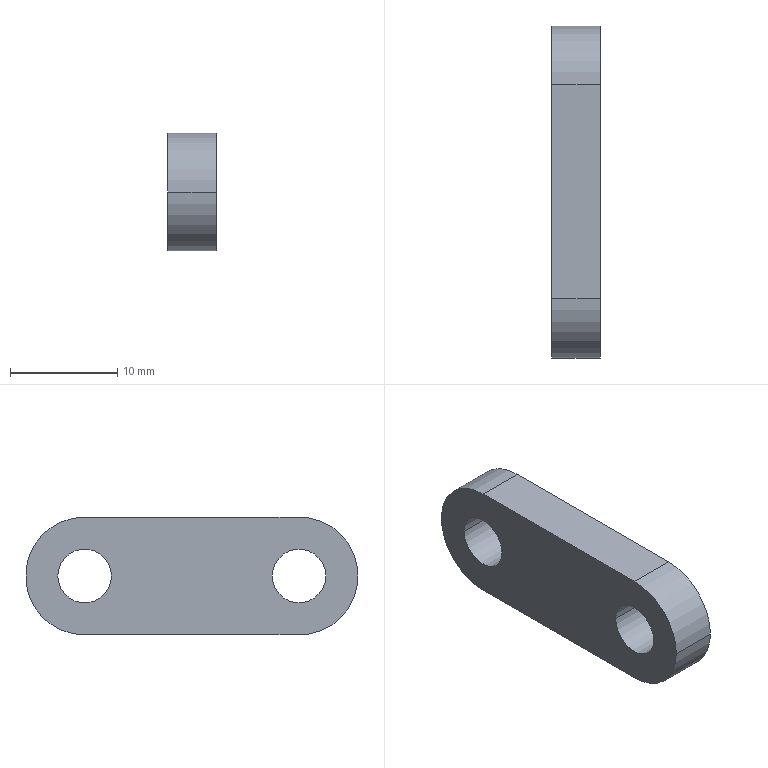Component | SolidWorks | LeverHydraulicRod22-1_HLKA-22_-0-2 | 1 solid | 11 faces | box 4.5 x 31 x 11 mm | volume 1241 mm3 | cylinder 7 | plane 4 | commonest cylinder face diameters 5 x4 11 x3
STEP:
#1=CARTESIAN_POINT('',(-2.288,4.392,-3.051));
#2=VERTEX_POINT('',#1);
#3=CARTESIAN_POINT('',(-2.288,4.588,-3.051));
#4=VERTEX_POINT('',#3);
#5=CARTESIAN_POINT('',(-2.288,4.49,-3.051));
#6=DIRECTION('',(1.,0.,0.));
#7=DIRECTION('',(0.,1.,0.));
#8=AXIS2_PLACEMENT_3D('',#5,#6,#7);
#9=CIRCLE('',#8,0.09843);
#10=EDGE_CURVE('',#2,#4,#9,.T.);
#11=ORIENTED_EDGE('',*,*,#10,.T.);
#12=CARTESIAN_POINT('',(-2.465,4.588,-3.051));
#13=VERTEX_POINT('',#12);
#14=CARTESIAN_POINT('',(-2.288,4.588,-3.051));
#15=DIRECTION('',(-1.,-0.,-0.));
#16=VECTOR('',#15,39.37);
#17=LINE('',#14,#16);
#18=EDGE_CURVE('',#4,#13,#17,.T.);
#19=ORIENTED_EDGE('',*,*,#18,.T.);
#20=CARTESIAN_POINT('',(-2.465,4.392,-3.051));
#21=VERTEX_POINT('',#20);
#22=CARTESIAN_POINT('',(-2.465,4.49,-3.051));
#23=DIRECTION('',(1.,0.,0.));
#24=DIRECTION('',(0.,1.,0.));
#25=AXIS2_PLACEMENT_3D('',#22,#23,#24);
#26=CIRCLE('',#25,0.09843);
#27=EDGE_CURVE('',#21,#13,#26,.T.);
#28=ORIENTED_EDGE('',*,*,#27,.F.);
#29=CARTESIAN_POINT('',(-2.288,4.392,-3.051));
#30=DIRECTION('',(-1.,-0.,-0.));
#31=VECTOR('',#30,39.37);
#32=LINE('',#29,#31);
#33=EDGE_CURVE('',#2,#21,#32,.T.);
#34=ORIENTED_EDGE('',*,*,#33,.F.);
#35=EDGE_LOOP('',(#11,#19,#28,#34));
#36=FACE_OUTER_BOUND('',#35,.T.);
#37=CARTESIAN_POINT('',(-2.288,4.49,-3.051));
#38=DIRECTION('',(-1.,-0.,-0.));
#39=DIRECTION('',(0.,-1.,0.));
#40=AXIS2_PLACEMENT_3D('',#37,#38,#39);
#41=CYLINDRICAL_SURFACE('',#40,0.09843);
#42=ADVANCED_FACE('',(#36),#41,.F.);
#43=CARTESIAN_POINT('',(-2.288,3.604,-3.051));
#44=VERTEX_POINT('',#43);
#45=CARTESIAN_POINT('',(-2.288,3.801,-3.051));
#46=VERTEX_POINT('',#45);
#47=CARTESIAN_POINT('',(-2.288,3.703,-3.051));
#48=DIRECTION('',(1.,0.,0.));
#49=DIRECTION('',(0.,1.,0.));
#50=AXIS2_PLACEMENT_3D('',#47,#48,#49);
#51=CIRCLE('',#50,0.09843);
#52=EDGE_CURVE('',#44,#46,#51,.T.);
#53=ORIENTED_EDGE('',*,*,#52,.T.);
#54=CARTESIAN_POINT('',(-2.465,3.801,-3.051));
#55=VERTEX_POINT('',#54);
#56=CARTESIAN_POINT('',(-2.288,3.801,-3.051));
#57=DIRECTION('',(-1.,-0.,-0.));
#58=VECTOR('',#57,39.37);
#59=LINE('',#56,#58);
#60=EDGE_CURVE('',#46,#55,#59,.T.);
#61=ORIENTED_EDGE('',*,*,#60,.T.);
#62=CARTESIAN_POINT('',(-2.465,3.604,-3.051));
#63=VERTEX_POINT('',#62);
#64=CARTESIAN_POINT('',(-2.465,3.703,-3.051));
#65=DIRECTION('',(1.,0.,0.));
#66=DIRECTION('',(0.,1.,0.));
#67=AXIS2_PLACEMENT_3D('',#64,#65,#66);
#68=CIRCLE('',#67,0.09843);
#69=EDGE_CURVE('',#63,#55,#68,.T.);
#70=ORIENTED_EDGE('',*,*,#69,.F.);
#71=CARTESIAN_POINT('',(-2.288,3.604,-3.051));
#72=DIRECTION('',(-1.,-0.,-0.));
#73=VECTOR('',#72,39.37);
#74=LINE('',#71,#73);
#75=EDGE_CURVE('',#44,#63,#74,.T.);
#76=ORIENTED_EDGE('',*,*,#75,.F.);
#77=EDGE_LOOP('',(#53,#61,#70,#76));
#78=FACE_OUTER_BOUND('',#77,.T.);
#79=CARTESIAN_POINT('',(-2.288,3.703,-3.051));
#80=DIRECTION('',(-1.,-0.,-0.));
#81=DIRECTION('',(0.,-1.,0.));
#82=AXIS2_PLACEMENT_3D('',#79,#80,#81);
#83=CYLINDRICAL_SURFACE('',#82,0.09843);
#84=ADVANCED_FACE('',(#78),#83,.F.);
#85=CARTESIAN_POINT('',(-2.288,3.486,-3.051));
#86=VERTEX_POINT('',#85);
#87=CARTESIAN_POINT('',(-2.288,3.703,-3.268));
#88=VERTEX_POINT('',#87);
#89=CARTESIAN_POINT('',(-2.288,3.703,-3.051));
#90=DIRECTION('',(1.,0.,0.));
#91=DIRECTION('',(0.,1.,0.));
#92=AXIS2_PLACEMENT_3D('',#89,#90,#91);
#93=CIRCLE('',#92,0.2165);
#94=EDGE_CURVE('',#86,#88,#93,.T.);
#95=ORIENTED_EDGE('',*,*,#94,.F.);
#96=CARTESIAN_POINT('',(-2.465,3.486,-3.051));
#97=VERTEX_POINT('',#96);
#98=CARTESIAN_POINT('',(-2.288,3.486,-3.051));
#99=DIRECTION('',(-1.,-0.,-0.));
#100=VECTOR('',#99,39.37);
#101=LINE('',#98,#100);
#102=EDGE_CURVE('',#86,#97,#101,.T.);
#103=ORIENTED_EDGE('',*,*,#102,.T.);
#104=CARTESIAN_POINT('',(-2.465,3.703,-3.268));
#105=VERTEX_POINT('',#104);
#106=CARTESIAN_POINT('',(-2.465,3.703,-3.051));
#107=DIRECTION('',(1.,0.,0.));
#108=DIRECTION('',(0.,1.,0.));
#109=AXIS2_PLACEMENT_3D('',#106,#107,#108);
#110=CIRCLE('',#109,0.2165);
#111=EDGE_CURVE('',#97,#105,#110,.T.);
#112=ORIENTED_EDGE('',*,*,#111,.T.);
#113=CARTESIAN_POINT('',(-2.288,3.703,-3.268));
#114=DIRECTION('',(-1.,-0.,-0.));
#115=VECTOR('',#114,39.37);
#116=LINE('',#113,#115);
#117=EDGE_CURVE('',#88,#105,#116,.T.);
#118=ORIENTED_EDGE('',*,*,#117,.F.);
#119=EDGE_LOOP('',(#95,#103,#112,#118));
#120=FACE_OUTER_BOUND('',#119,.T.);
#121=CARTESIAN_POINT('',(-2.288,3.703,-3.051));
#122=DIRECTION('',(-1.,-0.,-0.));
#123=DIRECTION('',(0.,-1.,0.));
#124=AXIS2_PLACEMENT_3D('',#121,#122,#123);
#125=CYLINDRICAL_SURFACE('',#124,0.2165);
#126=ADVANCED_FACE('',(#120),#125,.T.);
#127=CARTESIAN_POINT('',(-2.465,4.49,-2.835));
#128=VERTEX_POINT('',#127);
#129=CARTESIAN_POINT('',(-2.465,3.703,-2.835));
#130=VERTEX_POINT('',#129);
#131=CARTESIAN_POINT('',(-2.465,3.703,-2.835));
#132=DIRECTION('',(-0.,-1.,0.));
#133=VECTOR('',#132,39.37);
#134=LINE('',#131,#133);
#135=EDGE_CURVE('',#128,#130,#134,.T.);
#136=ORIENTED_EDGE('',*,*,#135,.T.);
#137=CARTESIAN_POINT('',(-2.288,3.703,-2.835));
#138=VERTEX_POINT('',#137);
#139=CARTESIAN_POINT('',(-2.288,3.703,-2.835));
#140=DIRECTION('',(-1.,-0.,-0.));
#141=VECTOR('',#140,39.37);
#142=LINE('',#139,#141);
#143=EDGE_CURVE('',#138,#130,#142,.T.);
#144=ORIENTED_EDGE('',*,*,#143,.F.);
#145=CARTESIAN_POINT('',(-2.288,4.49,-2.835));
#146=VERTEX_POINT('',#145);
#147=CARTESIAN_POINT('',(-2.288,3.703,-2.835));
#148=DIRECTION('',(-0.,-1.,0.));
#149=VECTOR('',#148,39.37);
#150=LINE('',#147,#149);
#151=EDGE_CURVE('',#146,#138,#150,.T.);
#152=ORIENTED_EDGE('',*,*,#151,.F.);
#153=CARTESIAN_POINT('',(-2.288,4.49,-2.835));
#154=DIRECTION('',(-1.,-0.,-0.));
#155=VECTOR('',#154,39.37);
#156=LINE('',#153,#155);
#157=EDGE_CURVE('',#146,#128,#156,.T.);
#158=ORIENTED_EDGE('',*,*,#157,.T.);
#159=EDGE_LOOP('',(#136,#144,#152,#158));
#160=FACE_OUTER_BOUND('',#159,.T.);
#161=CARTESIAN_POINT('',(-2.288,3.703,-2.835));
#162=DIRECTION('',(0.,-0.,-1.));
#163=DIRECTION('',(-1.,-0.,-0.));
#164=AXIS2_PLACEMENT_3D('',#161,#162,#163);
#165=PLANE('',#164);
#166=ADVANCED_FACE('',(#160),#165,.F.);
#167=CARTESIAN_POINT('',(-2.465,4.49,-3.268));
#168=VERTEX_POINT('',#167);
#169=CARTESIAN_POINT('',(-2.465,4.49,-3.051));
#170=DIRECTION('',(1.,0.,0.));
#171=DIRECTION('',(0.,1.,0.));
#172=AXIS2_PLACEMENT_3D('',#169,#170,#171);
#173=CIRCLE('',#172,0.2165);
#174=EDGE_CURVE('',#168,#128,#173,.T.);
#175=ORIENTED_EDGE('',*,*,#174,.T.);
#176=ORIENTED_EDGE('',*,*,#157,.F.);
#177=CARTESIAN_POINT('',(-2.288,4.49,-3.268));
#178=VERTEX_POINT('',#177);
#179=CARTESIAN_POINT('',(-2.288,4.49,-3.051));
#180=DIRECTION('',(1.,0.,0.));
#181=DIRECTION('',(0.,1.,0.));
#182=AXIS2_PLACEMENT_3D('',#179,#180,#181);
#183=CIRCLE('',#182,0.2165);
#184=EDGE_CURVE('',#178,#146,#183,.T.);
#185=ORIENTED_EDGE('',*,*,#184,.F.);
#186=CARTESIAN_POINT('',(-2.288,4.49,-3.268));
#187=DIRECTION('',(-1.,-0.,-0.));
#188=VECTOR('',#187,39.37);
#189=LINE('',#186,#188);
#190=EDGE_CURVE('',#178,#168,#189,.T.);
#191=ORIENTED_EDGE('',*,*,#190,.T.);
#192=EDGE_LOOP('',(#175,#176,#185,#191));
#193=FACE_OUTER_BOUND('',#192,.T.);
#194=CARTESIAN_POINT('',(-2.288,4.49,-3.051));
#195=DIRECTION('',(-1.,-0.,-0.));
#196=DIRECTION('',(0.,-1.,0.));
#197=AXIS2_PLACEMENT_3D('',#194,#195,#196);
#198=CYLINDRICAL_SURFACE('',#197,0.2165);
#199=ADVANCED_FACE('',(#193),#198,.T.);
#200=CARTESIAN_POINT('',(-2.465,3.703,-3.268));
#201=DIRECTION('',(0.,1.,-0.));
#202=VECTOR('',#201,39.37);
#203=LINE('',#200,#202);
#204=EDGE_CURVE('',#105,#168,#203,.T.);
#205=ORIENTED_EDGE('',*,*,#204,.T.);
#206=ORIENTED_EDGE('',*,*,#190,.F.);
#207=CARTESIAN_POINT('',(-2.288,3.703,-3.268));
#208=DIRECTION('',(0.,1.,-0.));
#209=VECTOR('',#208,39.37);
#210=LINE('',#207,#209);
#211=EDGE_CURVE('',#88,#178,#210,.T.);
#212=ORIENTED_EDGE('',*,*,#211,.F.);
#213=ORIENTED_EDGE('',*,*,#117,.T.);
#214=EDGE_LOOP('',(#205,#206,#212,#213));
#215=FACE_OUTER_BOUND('',#214,.T.);
#216=CARTESIAN_POINT('',(-2.288,3.703,-3.268));
#217=DIRECTION('',(-0.,0.,1.));
#218=DIRECTION('',(0.,1.,-0.));
#219=AXIS2_PLACEMENT_3D('',#216,#217,#218);
#220=PLANE('',#219);
#221=ADVANCED_FACE('',(#215),#220,.F.);
#222=ORIENTED_EDGE('',*,*,#27,.T.);
#223=CARTESIAN_POINT('',(-2.465,4.49,-3.051));
#224=DIRECTION('',(1.,0.,0.));
#225=DIRECTION('',(0.,1.,0.));
#226=AXIS2_PLACEMENT_3D('',#223,#224,#225);
#227=CIRCLE('',#226,0.09843);
#228=EDGE_CURVE('',#13,#21,#227,.T.);
#229=ORIENTED_EDGE('',*,*,#228,.T.);
#230=EDGE_LOOP('',(#222,#229));
#231=FACE_BOUND('',#230,.T.);
#232=ORIENTED_EDGE('',*,*,#69,.T.);
#233=CARTESIAN_POINT('',(-2.465,3.703,-3.051));
#234=DIRECTION('',(1.,0.,0.));
#235=DIRECTION('',(0.,1.,0.));
#236=AXIS2_PLACEMENT_3D('',#233,#234,#235);
#237=CIRCLE('',#236,0.09843);
#238=EDGE_CURVE('',#55,#63,#237,.T.);
#239=ORIENTED_EDGE('',*,*,#238,.T.);
#240=EDGE_LOOP('',(#232,#239));
#241=FACE_BOUND('',#240,.T.);
#242=CARTESIAN_POINT('',(-2.465,3.703,-3.051));
#243=DIRECTION('',(1.,0.,0.));
#244=DIRECTION('',(0.,1.,0.));
#245=AXIS2_PLACEMENT_3D('',#242,#243,#244);
#246=CIRCLE('',#245,0.2165);
#247=EDGE_CURVE('',#130,#97,#246,.T.);
#248=ORIENTED_EDGE('',*,*,#247,.F.);
#249=ORIENTED_EDGE('',*,*,#135,.F.);
#250=ORIENTED_EDGE('',*,*,#174,.F.);
#251=ORIENTED_EDGE('',*,*,#204,.F.);
#252=ORIENTED_EDGE('',*,*,#111,.F.);
#253=EDGE_LOOP('',(#248,#249,#250,#251,#252));
#254=FACE_OUTER_BOUND('',#253,.T.);
#255=CARTESIAN_POINT('',(-2.465,3.703,-3.051));
#256=DIRECTION('',(1.,0.,0.));
#257=DIRECTION('',(0.,1.,-0.));
#258=AXIS2_PLACEMENT_3D('',#255,#256,#257);
#259=PLANE('',#258);
#260=ADVANCED_FACE('',(#231,#241,#254),#259,.F.);
#261=ORIENTED_EDGE('',*,*,#10,.F.);
#262=CARTESIAN_POINT('',(-2.288,4.49,-3.051));
#263=DIRECTION('',(1.,0.,0.));
#264=DIRECTION('',(0.,1.,0.));
#265=AXIS2_PLACEMENT_3D('',#262,#263,#264);
#266=CIRCLE('',#265,0.09843);
#267=EDGE_CURVE('',#4,#2,#266,.T.);
#268=ORIENTED_EDGE('',*,*,#267,.F.);
#269=EDGE_LOOP('',(#261,#268));
#270=FACE_BOUND('',#269,.T.);
#271=ORIENTED_EDGE('',*,*,#52,.F.);
#272=CARTESIAN_POINT('',(-2.288,3.703,-3.051));
#273=DIRECTION('',(1.,0.,0.));
#274=DIRECTION('',(0.,1.,0.));
#275=AXIS2_PLACEMENT_3D('',#272,#273,#274);
#276=CIRCLE('',#275,0.09843);
#277=EDGE_CURVE('',#46,#44,#276,.T.);
#278=ORIENTED_EDGE('',*,*,#277,.F.);
#279=EDGE_LOOP('',(#271,#278));
#280=FACE_BOUND('',#279,.T.);
#281=ORIENTED_EDGE('',*,*,#151,.T.);
#282=CARTESIAN_POINT('',(-2.288,3.703,-3.051));
#283=DIRECTION('',(1.,0.,0.));
#284=DIRECTION('',(0.,1.,0.));
#285=AXIS2_PLACEMENT_3D('',#282,#283,#284);
#286=CIRCLE('',#285,0.2165);
#287=EDGE_CURVE('',#138,#86,#286,.T.);
#288=ORIENTED_EDGE('',*,*,#287,.T.);
#289=ORIENTED_EDGE('',*,*,#94,.T.);
#290=ORIENTED_EDGE('',*,*,#211,.T.);
#291=ORIENTED_EDGE('',*,*,#184,.T.);
#292=EDGE_LOOP('',(#281,#288,#289,#290,#291));
#293=FACE_OUTER_BOUND('',#292,.T.);
#294=CARTESIAN_POINT('',(-2.288,3.703,-3.051));
#295=DIRECTION('',(1.,0.,0.));
#296=DIRECTION('',(0.,1.,-0.));
#297=AXIS2_PLACEMENT_3D('',#294,#295,#296);
#298=PLANE('',#297);
#299=ADVANCED_FACE('',(#270,#280,#293),#298,.T.);
#300=ORIENTED_EDGE('',*,*,#102,.F.);
#301=ORIENTED_EDGE('',*,*,#287,.F.);
#302=ORIENTED_EDGE('',*,*,#143,.T.);
#303=ORIENTED_EDGE('',*,*,#247,.T.);
#304=EDGE_LOOP('',(#300,#301,#302,#303));
#305=FACE_OUTER_BOUND('',#304,.T.);
#306=CARTESIAN_POINT('',(-2.288,3.703,-3.051));
#307=DIRECTION('',(-1.,-0.,-0.));
#308=DIRECTION('',(0.,-1.,0.));
#309=AXIS2_PLACEMENT_3D('',#306,#307,#308);
#310=CYLINDRICAL_SURFACE('',#309,0.2165);
#311=ADVANCED_FACE('',(#305),#310,.T.);
#312=ORIENTED_EDGE('',*,*,#60,.F.);
#313=ORIENTED_EDGE('',*,*,#277,.T.);
#314=ORIENTED_EDGE('',*,*,#75,.T.);
#315=ORIENTED_EDGE('',*,*,#238,.F.);
#316=EDGE_LOOP('',(#312,#313,#314,#315));
#317=FACE_OUTER_BOUND('',#316,.T.);
#318=CARTESIAN_POINT('',(-2.288,3.703,-3.051));
#319=DIRECTION('',(-1.,-0.,-0.));
#320=DIRECTION('',(0.,-1.,0.));
#321=AXIS2_PLACEMENT_3D('',#318,#319,#320);
#322=CYLINDRICAL_SURFACE('',#321,0.09843);
#323=ADVANCED_FACE('',(#317),#322,.F.);
#324=ORIENTED_EDGE('',*,*,#18,.F.);
#325=ORIENTED_EDGE('',*,*,#267,.T.);
#326=ORIENTED_EDGE('',*,*,#33,.T.);
#327=ORIENTED_EDGE('',*,*,#228,.F.);
#328=EDGE_LOOP('',(#324,#325,#326,#327));
#329=FACE_OUTER_BOUND('',#328,.T.);
#330=CARTESIAN_POINT('',(-2.288,4.49,-3.051));
#331=DIRECTION('',(-1.,-0.,-0.));
#332=DIRECTION('',(0.,-1.,0.));
#333=AXIS2_PLACEMENT_3D('',#330,#331,#332);
#334=CYLINDRICAL_SURFACE('',#333,0.09843);
#335=ADVANCED_FACE('',(#329),#334,.F.);
#336=CLOSED_SHELL('',(#42,#84,#126,#166,#199,#221,#260,#299,#311,#323,#335));
#337=MANIFOLD_SOLID_BREP('',#336);
#338=CARTESIAN_POINT('',(0.,0.,0.));
#339=DIRECTION('',(0.,0.,1.));
#340=DIRECTION('',(1.,0.,0.));
#341=AXIS2_PLACEMENT_3D('',#338,#339,#340);
#342=(LENGTH_UNIT()NAMED_UNIT(*)SI_UNIT($,.METRE.));
#343=LENGTH_MEASURE_WITH_UNIT(LENGTH_MEASURE(0.0254),#342);
#344=DIMENSIONAL_EXPONENTS(1.,0.,0.,0.,0.,0.,0.);
#345=(CONVERSION_BASED_UNIT('',#343)LENGTH_UNIT()NAMED_UNIT(#344));
#346=UNCERTAINTY_MEASURE_WITH_UNIT(LENGTH_MEASURE(0.00001),#345,'','');
#347=(NAMED_UNIT(*)PLANE_ANGLE_UNIT()SI_UNIT($,.RADIAN.));
#348=(NAMED_UNIT(*)SI_UNIT($,.STERADIAN.)SOLID_ANGLE_UNIT());
#349=(GEOMETRIC_REPRESENTATION_CONTEXT(3)GLOBAL_UNCERTAINTY_ASSIGNED_CONTEXT((#346))GLOBAL_UNIT_ASSIGNED_CONTEXT((#345,#347,#348))REPRESENTATION_CONTEXT('',''));
#350=ADVANCED_BREP_SHAPE_REPRESENTATION('',(#337,#341),#349);
#351=COLOUR_RGB('',0.7922,0.8196,0.9333);
#352=FILL_AREA_STYLE_COLOUR('',#351);
#353=FILL_AREA_STYLE('',(#352));
#354=SURFACE_STYLE_FILL_AREA(#353);
#355=SURFACE_SIDE_STYLE('',(#354));
#356=SURFACE_STYLE_USAGE(.BOTH.,#355);
#357=PRESENTATION_STYLE_ASSIGNMENT((#356));
#358=STYLED_ITEM('',(#357),#337);
#359=PRESENTATION_LAYER_ASSIGNMENT('','',(#358));
#360=(LENGTH_UNIT()NAMED_UNIT(*)SI_UNIT($,.METRE.));
#361=LENGTH_MEASURE_WITH_UNIT(LENGTH_MEASURE(0.0254),#360);
#362=DIMENSIONAL_EXPONENTS(1.,0.,0.,0.,0.,0.,0.);
#363=(CONVERSION_BASED_UNIT('',#361)LENGTH_UNIT()NAMED_UNIT(#362));
#364=UNCERTAINTY_MEASURE_WITH_UNIT(LENGTH_MEASURE(0.00001),#363,'','');
#365=(NAMED_UNIT(*)PLANE_ANGLE_UNIT()SI_UNIT($,.RADIAN.));
#366=(NAMED_UNIT(*)SI_UNIT($,.STERADIAN.)SOLID_ANGLE_UNIT());
#367=(GEOMETRIC_REPRESENTATION_CONTEXT(3)GLOBAL_UNCERTAINTY_ASSIGNED_CONTEXT((#364))GLOBAL_UNIT_ASSIGNED_CONTEXT((#363,#365,#366))REPRESENTATION_CONTEXT('',''));
#368=MECHANICAL_DESIGN_GEOMETRIC_PRESENTATION_REPRESENTATION('',(#358),#367);